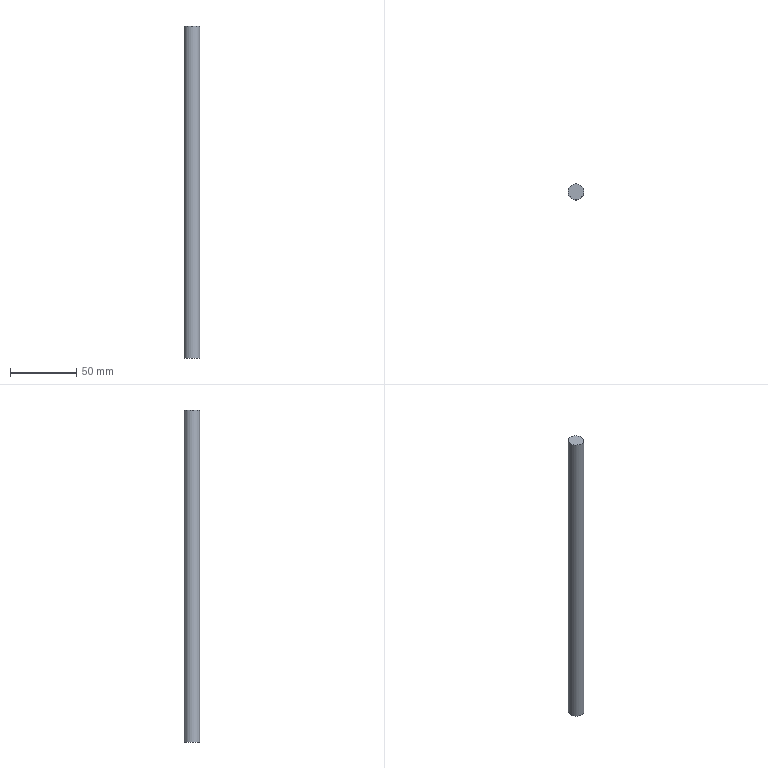Component | NX | SMOOTH_SHAFT_2 | 1 solid | 3 faces | box 12 x 12 x 250 mm | volume 28274 mm3 | plane 2 | cylinder 1 | commonest cylinder face diameters 12 x1
STEP:
#1=CARTESIAN_POINT('',(0.,0.,0.));
#2=DIRECTION('',(0.,0.,1.));
#3=DIRECTION('',(1.,0.,0.));
#4=AXIS2_PLACEMENT_3D('',#1,#2,#3);
#5=CARTESIAN_POINT('',(6.,0.,237.));
#6=VERTEX_POINT('',#5);
#7=CARTESIAN_POINT('',(0.,0.,237.));
#8=DIRECTION('',(0.,0.,-1.));
#9=DIRECTION('',(1.,0.,0.));
#10=AXIS2_PLACEMENT_3D('',#7,#8,#9);
#11=CIRCLE('',#10,6.);
#12=CARTESIAN_POINT('',(0.,0.,237.));
#13=DIRECTION('',(0.,0.,1.));
#14=DIRECTION('',(1.,0.,0.));
#15=AXIS2_PLACEMENT_3D('',#12,#13,#14);
#16=PLANE('',#15);
#17=CARTESIAN_POINT('',(6.,0.));
#18=CARTESIAN_POINT('',(6.,-10.392));
#19=CARTESIAN_POINT('',(-3.,-5.196));
#20=CARTESIAN_POINT('',(-12.,-0.));
#21=CARTESIAN_POINT('',(-3.,5.196));
#22=CARTESIAN_POINT('',(6.,10.392));
#23=CARTESIAN_POINT('',(6.,0.));
#24=(BOUNDED_CURVE()B_SPLINE_CURVE(2,(#17,#18,#19,#20,#21,#22,#23),.UNSPECIFIED.,.T.,.F.)B_SPLINE_CURVE_WITH_KNOTS((1,2,2,2,2,1),(-2.094,0.,2.094,4.189,6.283,8.378),.UNSPECIFIED.)CURVE()GEOMETRIC_REPRESENTATION_ITEM()RATIONAL_B_SPLINE_CURVE((1.,0.5,1.,0.5,1.,0.5,1.))REPRESENTATION_ITEM(''));
#25=(GEOMETRIC_REPRESENTATION_CONTEXT(2)PARAMETRIC_REPRESENTATION_CONTEXT()REPRESENTATION_CONTEXT('',''));
#26=DEFINITIONAL_REPRESENTATION('',(#24),#25);
#27=PCURVE('',#16,#26);
#28=CARTESIAN_POINT('',(0.,0.,-13.));
#29=DIRECTION('',(0.,0.,1.));
#30=DIRECTION('',(1.,0.,0.));
#31=AXIS2_PLACEMENT_3D('',#28,#29,#30);
#32=CYLINDRICAL_SURFACE('',#31,6.);
#33=CARTESIAN_POINT('',(6.283,250.));
#34=DIRECTION('',(-1.,0.));
#35=VECTOR('',#34,1.);
#36=LINE('',#33,#35);
#37=(GEOMETRIC_REPRESENTATION_CONTEXT(2)PARAMETRIC_REPRESENTATION_CONTEXT()REPRESENTATION_CONTEXT('',''));
#38=DEFINITIONAL_REPRESENTATION('',(#36),#37);
#39=PCURVE('',#32,#38);
#40=SURFACE_CURVE('',#11,(#27,#39),.PCURVE_S1.);
#41=EDGE_CURVE('',#6,#6,#40,.T.);
#42=ORIENTED_EDGE('',*,*,#41,.F.);
#43=EDGE_LOOP('',(#42));
#44=FACE_BOUND('',#43,.T.);
#45=ADVANCED_FACE('',(#44),#16,.T.);
#46=CARTESIAN_POINT('',(6.,0.,-13.));
#47=VERTEX_POINT('',#46);
#48=CARTESIAN_POINT('',(0.,0.,-13.));
#49=DIRECTION('',(0.,0.,1.));
#50=DIRECTION('',(1.,0.,0.));
#51=AXIS2_PLACEMENT_3D('',#48,#49,#50);
#52=CIRCLE('',#51,6.);
#53=CARTESIAN_POINT('',(0.,0.,-13.));
#54=DIRECTION('',(0.,0.,-1.));
#55=DIRECTION('',(-1.,0.,0.));
#56=AXIS2_PLACEMENT_3D('',#53,#54,#55);
#57=PLANE('',#56);
#58=CARTESIAN_POINT('',(-6.,0.));
#59=CARTESIAN_POINT('',(-6.,10.392));
#60=CARTESIAN_POINT('',(3.,5.196));
#61=CARTESIAN_POINT('',(12.,0.));
#62=CARTESIAN_POINT('',(3.,-5.196));
#63=CARTESIAN_POINT('',(-6.,-10.392));
#64=CARTESIAN_POINT('',(-6.,0.));
#65=(BOUNDED_CURVE()B_SPLINE_CURVE(2,(#58,#59,#60,#61,#62,#63,#64),.UNSPECIFIED.,.T.,.F.)B_SPLINE_CURVE_WITH_KNOTS((1,2,2,2,2,1),(-2.094,0.,2.094,4.189,6.283,8.378),.UNSPECIFIED.)CURVE()GEOMETRIC_REPRESENTATION_ITEM()RATIONAL_B_SPLINE_CURVE((1.,0.5,1.,0.5,1.,0.5,1.))REPRESENTATION_ITEM(''));
#66=(GEOMETRIC_REPRESENTATION_CONTEXT(2)PARAMETRIC_REPRESENTATION_CONTEXT()REPRESENTATION_CONTEXT('',''));
#67=DEFINITIONAL_REPRESENTATION('',(#65),#66);
#68=PCURVE('',#57,#67);
#69=CARTESIAN_POINT('',(0.,0.));
#70=DIRECTION('',(1.,0.));
#71=VECTOR('',#70,1.);
#72=LINE('',#69,#71);
#73=(GEOMETRIC_REPRESENTATION_CONTEXT(2)PARAMETRIC_REPRESENTATION_CONTEXT()REPRESENTATION_CONTEXT('',''));
#74=DEFINITIONAL_REPRESENTATION('',(#72),#73);
#75=PCURVE('',#32,#74);
#76=SURFACE_CURVE('',#52,(#68,#75),.PCURVE_S1.);
#77=EDGE_CURVE('',#47,#47,#76,.T.);
#78=ORIENTED_EDGE('',*,*,#77,.F.);
#79=EDGE_LOOP('',(#78));
#80=FACE_BOUND('',#79,.T.);
#81=ADVANCED_FACE('',(#80),#57,.T.);
#82=ORIENTED_EDGE('',*,*,#41,.T.);
#83=CARTESIAN_POINT('',(6.,-0.,-13.));
#84=CARTESIAN_POINT('',(6.,-0.,237.));
#85=B_SPLINE_CURVE_WITH_KNOTS('',1,(#83,#84),.UNSPECIFIED.,.F.,.F.,(2,2),(0.,250.),.PIECEWISE_BEZIER_KNOTS.);
#86=CARTESIAN_POINT('',(0.,0.));
#87=DIRECTION('',(0.,1.));
#88=VECTOR('',#87,1.);
#89=LINE('',#86,#88);
#90=(GEOMETRIC_REPRESENTATION_CONTEXT(2)PARAMETRIC_REPRESENTATION_CONTEXT()REPRESENTATION_CONTEXT('',''));
#91=DEFINITIONAL_REPRESENTATION('',(#89),#90);
#92=PCURVE('',#32,#91);
#93=CARTESIAN_POINT('',(6.283,0.));
#94=DIRECTION('',(0.,1.));
#95=VECTOR('',#94,1.);
#96=LINE('',#93,#95);
#97=(GEOMETRIC_REPRESENTATION_CONTEXT(2)PARAMETRIC_REPRESENTATION_CONTEXT()REPRESENTATION_CONTEXT('',''));
#98=DEFINITIONAL_REPRESENTATION('',(#96),#97);
#99=PCURVE('',#32,#98);
#100=SEAM_CURVE('',#85,(#92,#99),.PCURVE_S1.);
#101=EDGE_CURVE('',#47,#6,#100,.T.);
#102=ORIENTED_EDGE('',*,*,#101,.F.);
#103=ORIENTED_EDGE('',*,*,#77,.T.);
#104=ORIENTED_EDGE('',*,*,#101,.T.);
#105=EDGE_LOOP('',(#82,#102,#103,#104));
#106=FACE_BOUND('',#105,.T.);
#107=ADVANCED_FACE('',(#106),#32,.T.);
#108=CLOSED_SHELL('',(#45,#81,#107));
#109=MANIFOLD_SOLID_BREP('',#108);
#110=(LENGTH_UNIT()NAMED_UNIT(*)SI_UNIT(.MILLI.,.METRE.));
#111=UNCERTAINTY_MEASURE_WITH_UNIT(LENGTH_MEASURE(0.00001),#110,'','');
#112=(NAMED_UNIT(*)PLANE_ANGLE_UNIT()SI_UNIT($,.RADIAN.));
#113=(NAMED_UNIT(*)SI_UNIT($,.STERADIAN.)SOLID_ANGLE_UNIT());
#114=(GEOMETRIC_REPRESENTATION_CONTEXT(3)GLOBAL_UNCERTAINTY_ASSIGNED_CONTEXT((#111))GLOBAL_UNIT_ASSIGNED_CONTEXT((#110,#112,#113))REPRESENTATION_CONTEXT('',''));
#115=ADVANCED_BREP_SHAPE_REPRESENTATION('',(#4,#109),#114);